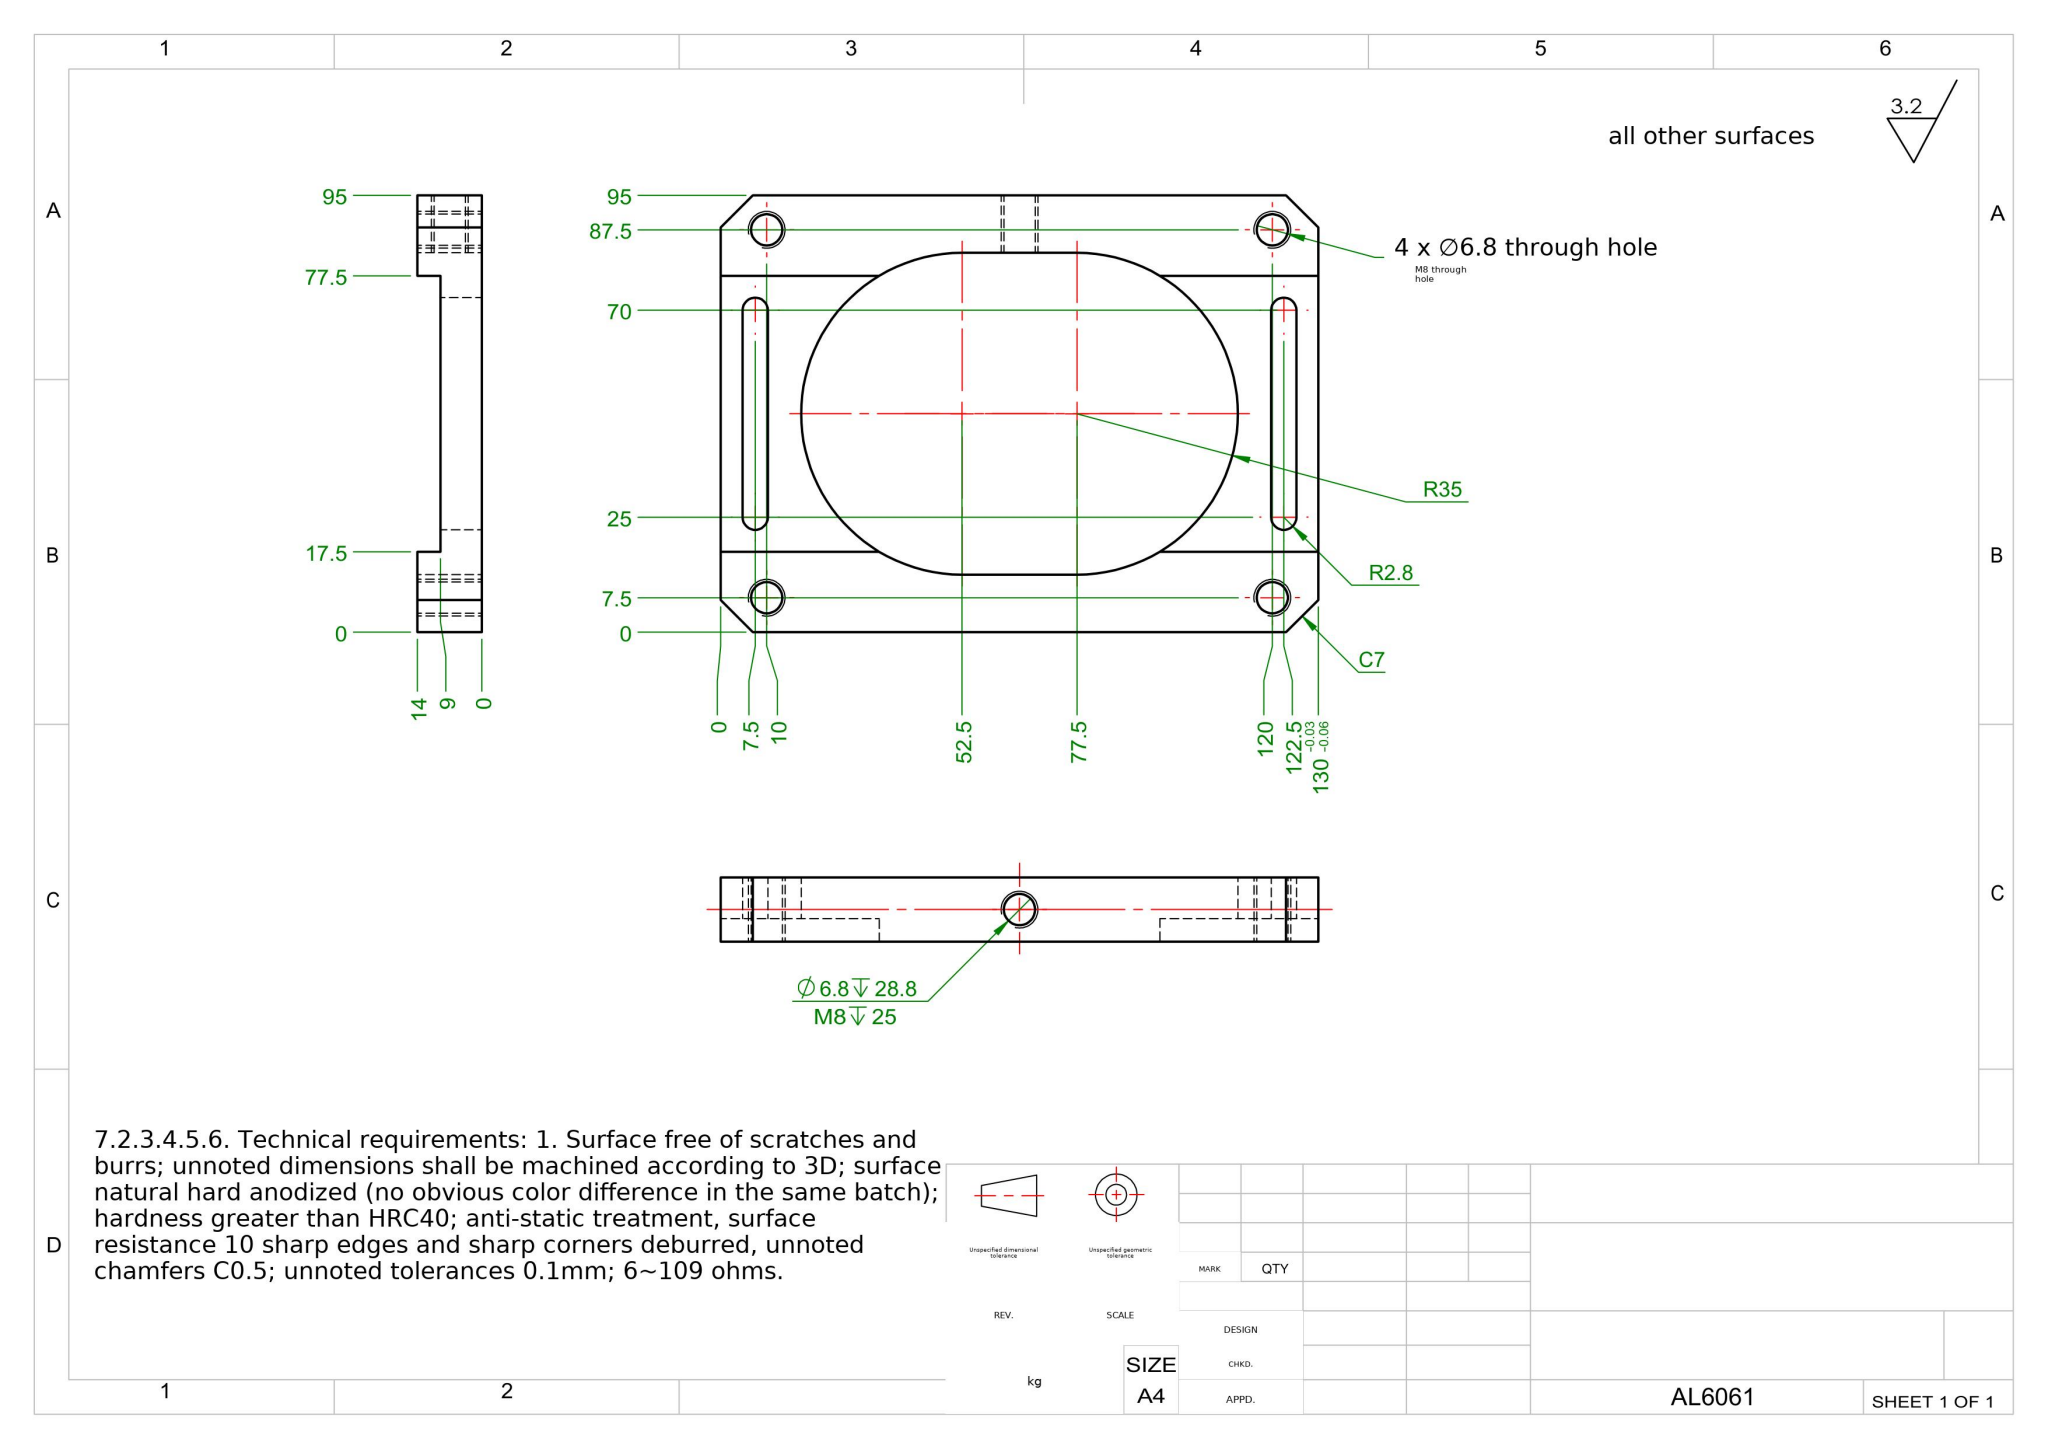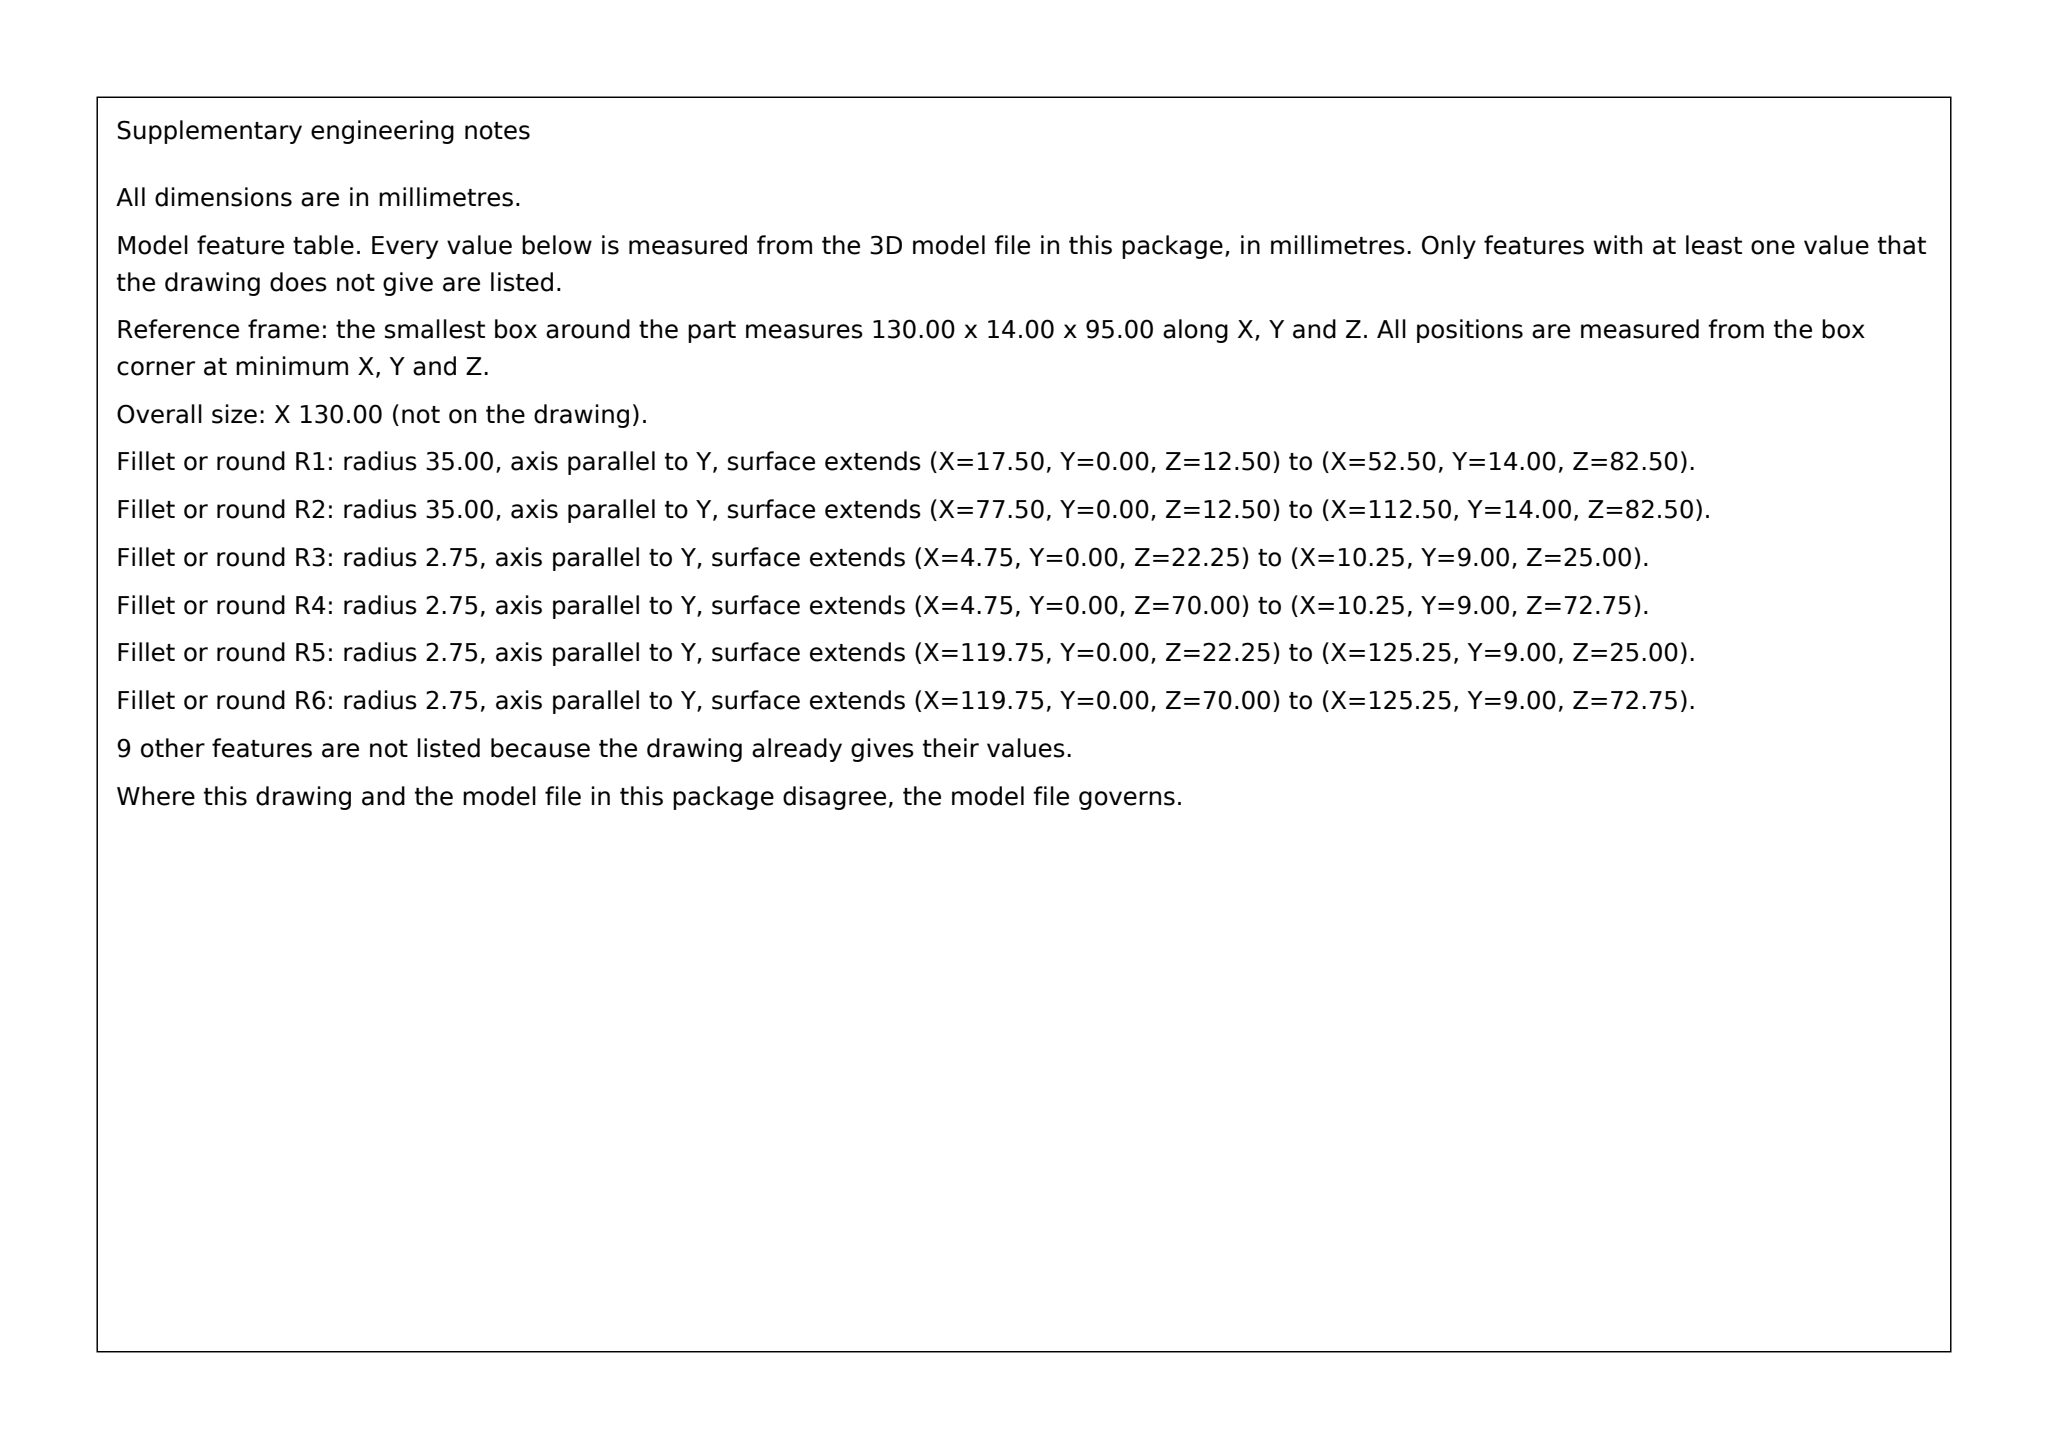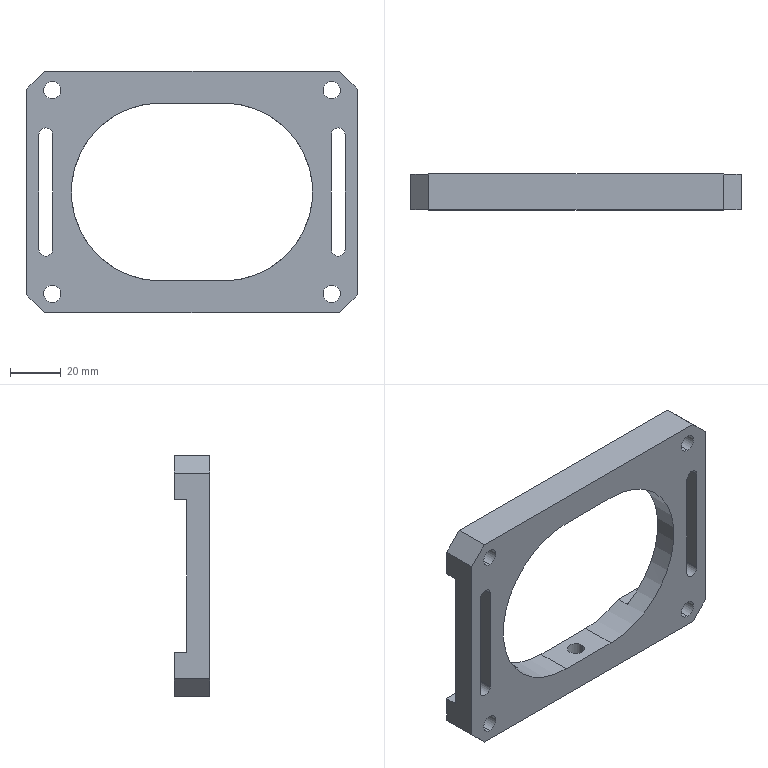Part | SolidWorks | mm | 1 solid | 41 faces | box 130 x 14 x 95 mm | volume 72301 mm3 | plane 23 | cylinder 18 | commonest cylinder face diameters 6.8 x10 5.5 x6 70 x2
build123d program:
from build123d import *

# Parameters (mm, degrees)
SKETCH1_W               = 130
SKETCH1_H               = 95
BOSS_EXTRUDE1_DEPTH     = 7
CUT_EXTRUDE1_DEPTH      = 82.714
CUT_EXTRUDE1_DEPTH_BACK = 82.714
CHAMFER1_SIZE           = 7
CUT_EXTRUDE2_DEPTH      = 82.714
M8_TAPPED_HOLE1_D       = 6.8
M8_TAPPED_HOLE1_DEPTH   = 28.75
M8_TAPPED_HOLE1_TIP     = 2.043
M8_TAPPED_HOLE2_D       = 6.8
SKETCH8_W               = 60
SKETCH8_H               = 10
CUT_EXTRUDE3_DEPTH      = 139.583


with BuildPart() as part:
    # Sketch1 → Boss-Extrude1 (new, symmetric)
    with BuildSketch(Plane(origin=(0, 0, 0), x_dir=(1, 0, 0), z_dir=(0, 1, 0))):
        Rectangle(SKETCH1_W, SKETCH1_H)
    extrude(amount=BOSS_EXTRUDE1_DEPTH, both=True)

    # Sketch2 → Cut-Extrude1 (cut, two sides: drawn at the far end of the back side and taken through both)
    with BuildSketch(Plane(origin=(0, 7, 0), x_dir=(1, 0, 0), z_dir=(0, 1, 0)).offset(-CUT_EXTRUDE1_DEPTH_BACK)):
        with BuildLine():
            Line((12.5, -35), (-12.5, -35))
            ThreePointArc((-12.5, -35), (-47.5, 0), (-12.5, 35))
            Line((-12.5, 35), (12.5, 35))
            ThreePointArc((12.5, 35), (47.5, 0), (12.5, -35))
        make_face()
    extrude(amount=CUT_EXTRUDE1_DEPTH + CUT_EXTRUDE1_DEPTH_BACK, mode=Mode.SUBTRACT)

    # Chamfer1
    chamfer1_edges = [part.edges().sort_by_distance(p)[0] for p in [
        (65, 0, 47.5),
        (-65, 0, 47.5),
        (-65, 0, -47.5),
        (65, 0, -47.5),
    ]]
    chamfer(chamfer1_edges, length=CHAMFER1_SIZE)

    # Sketch3 → Cut-Extrude2 (cut, through all)
    with BuildSketch(Plane(origin=(0, 7, 0), x_dir=(1, 0, 0), z_dir=(0, 1, 0))):
        with BuildLine():
            Line((-60.25, -22.5), (-60.25, 22.5))
            ThreePointArc((-60.25, 22.5), (-57.5, 25.25), (-54.75, 22.5))
            Line((-54.75, 22.5), (-54.75, -22.5))
            ThreePointArc((-54.75, -22.5), (-57.5, -25.25), (-60.25, -22.5))
        make_face()
        with BuildLine():
            Line((54.75, -22.5), (54.75, 22.5))
            ThreePointArc((54.75, 22.5), (57.5, 25.25), (60.25, 22.5))
            Line((60.25, 22.5), (60.25, -22.5))
            ThreePointArc((60.25, -22.5), (57.5, -25.25), (54.75, -22.5))
        make_face()
    extrude(amount=-CUT_EXTRUDE2_DEPTH, mode=Mode.SUBTRACT)

    # M8 Tapped Hole1
    with Locations(Plane(origin=(0, 0, -47.5), x_dir=(-1, 0, 0), z_dir=(0, 0, -1))):
        with Locations((0, 0)):
            Hole(M8_TAPPED_HOLE1_D / 2, depth=M8_TAPPED_HOLE1_DEPTH)
            with Locations((0, 0, -(M8_TAPPED_HOLE1_DEPTH + M8_TAPPED_HOLE1_TIP / 2))):  # 118° drill point
                Cone(0, M8_TAPPED_HOLE1_D / 2, M8_TAPPED_HOLE1_TIP, mode=Mode.SUBTRACT)

    # M8 Tapped Hole2 (through all)
    with Locations(Plane(origin=(0, 7, 0), x_dir=(1, 0, 0), z_dir=(0, 1, 0))):
        with Locations((-55, -40), (-55, 40), (55, -40), (55, 40)):
            Hole(M8_TAPPED_HOLE2_D / 2)

    # Sketch8 → Cut-Extrude3 (cut, through all)
    with BuildSketch(Plane.ZY.offset(65)):
        with Locations((0, 7)):
            Rectangle(SKETCH8_W, SKETCH8_H)
    extrude(amount=-CUT_EXTRUDE3_DEPTH, mode=Mode.SUBTRACT)


solid = part.part